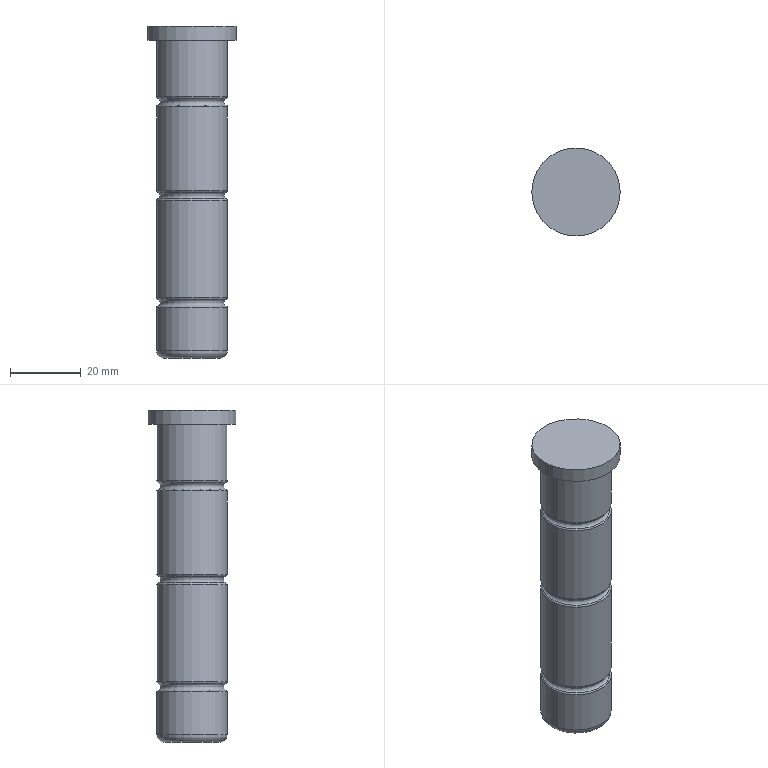Component | NX | PILLER_BUSH | 1 solid | 18 faces | volume 29935 mm3 | torus 10 | cylinder 5 | plane 3 | commonest cylinder face diameters 20.015 x4 25 x1